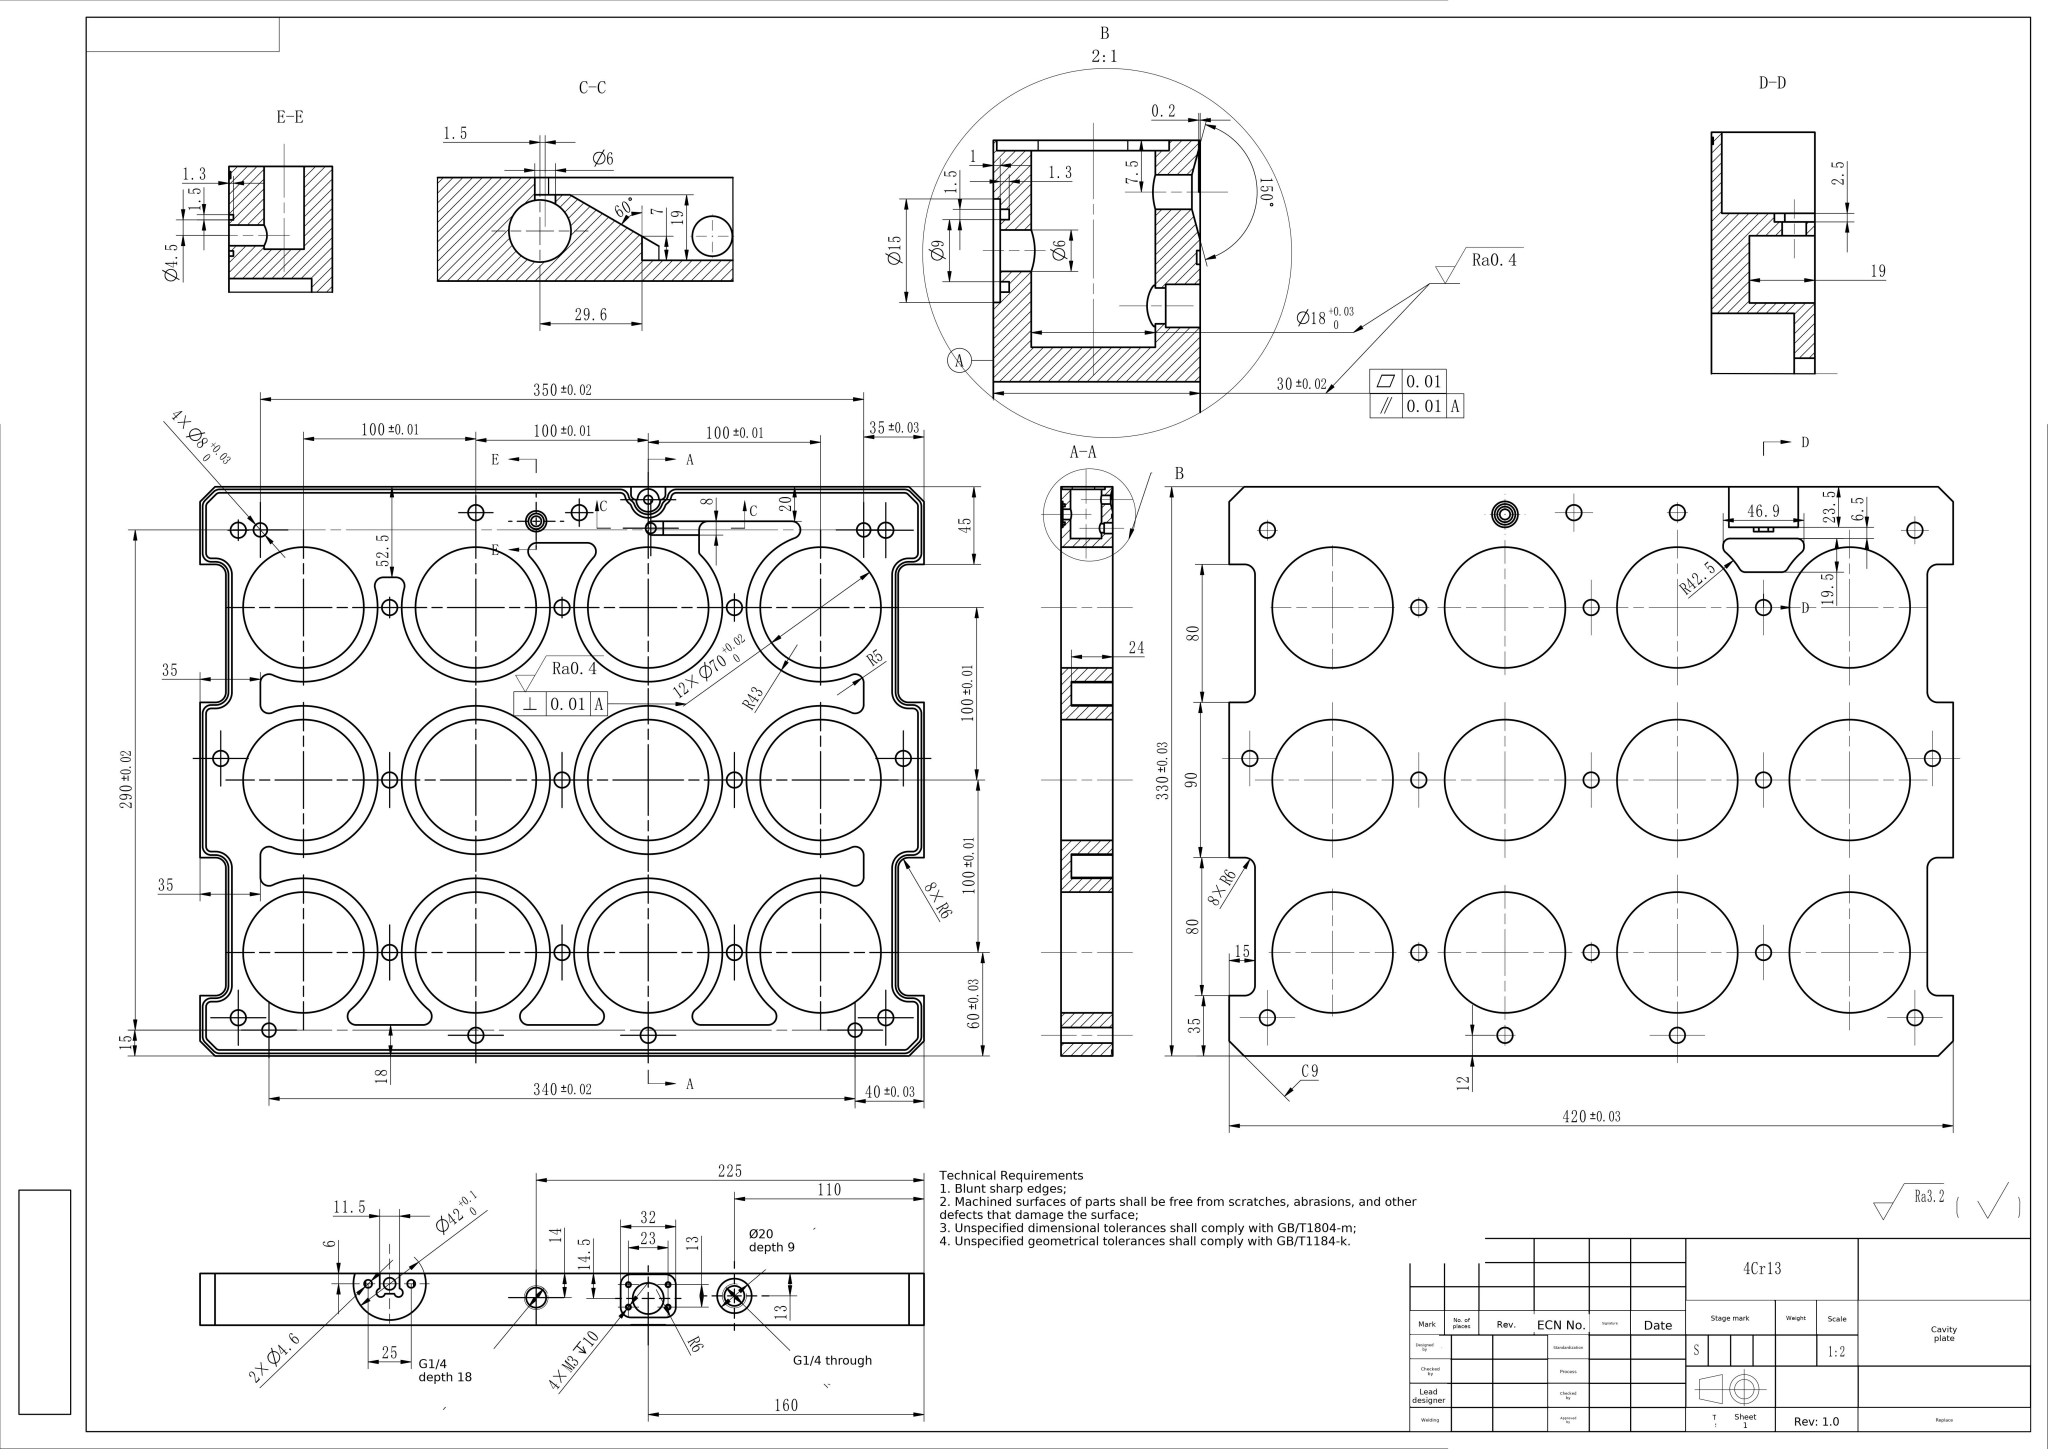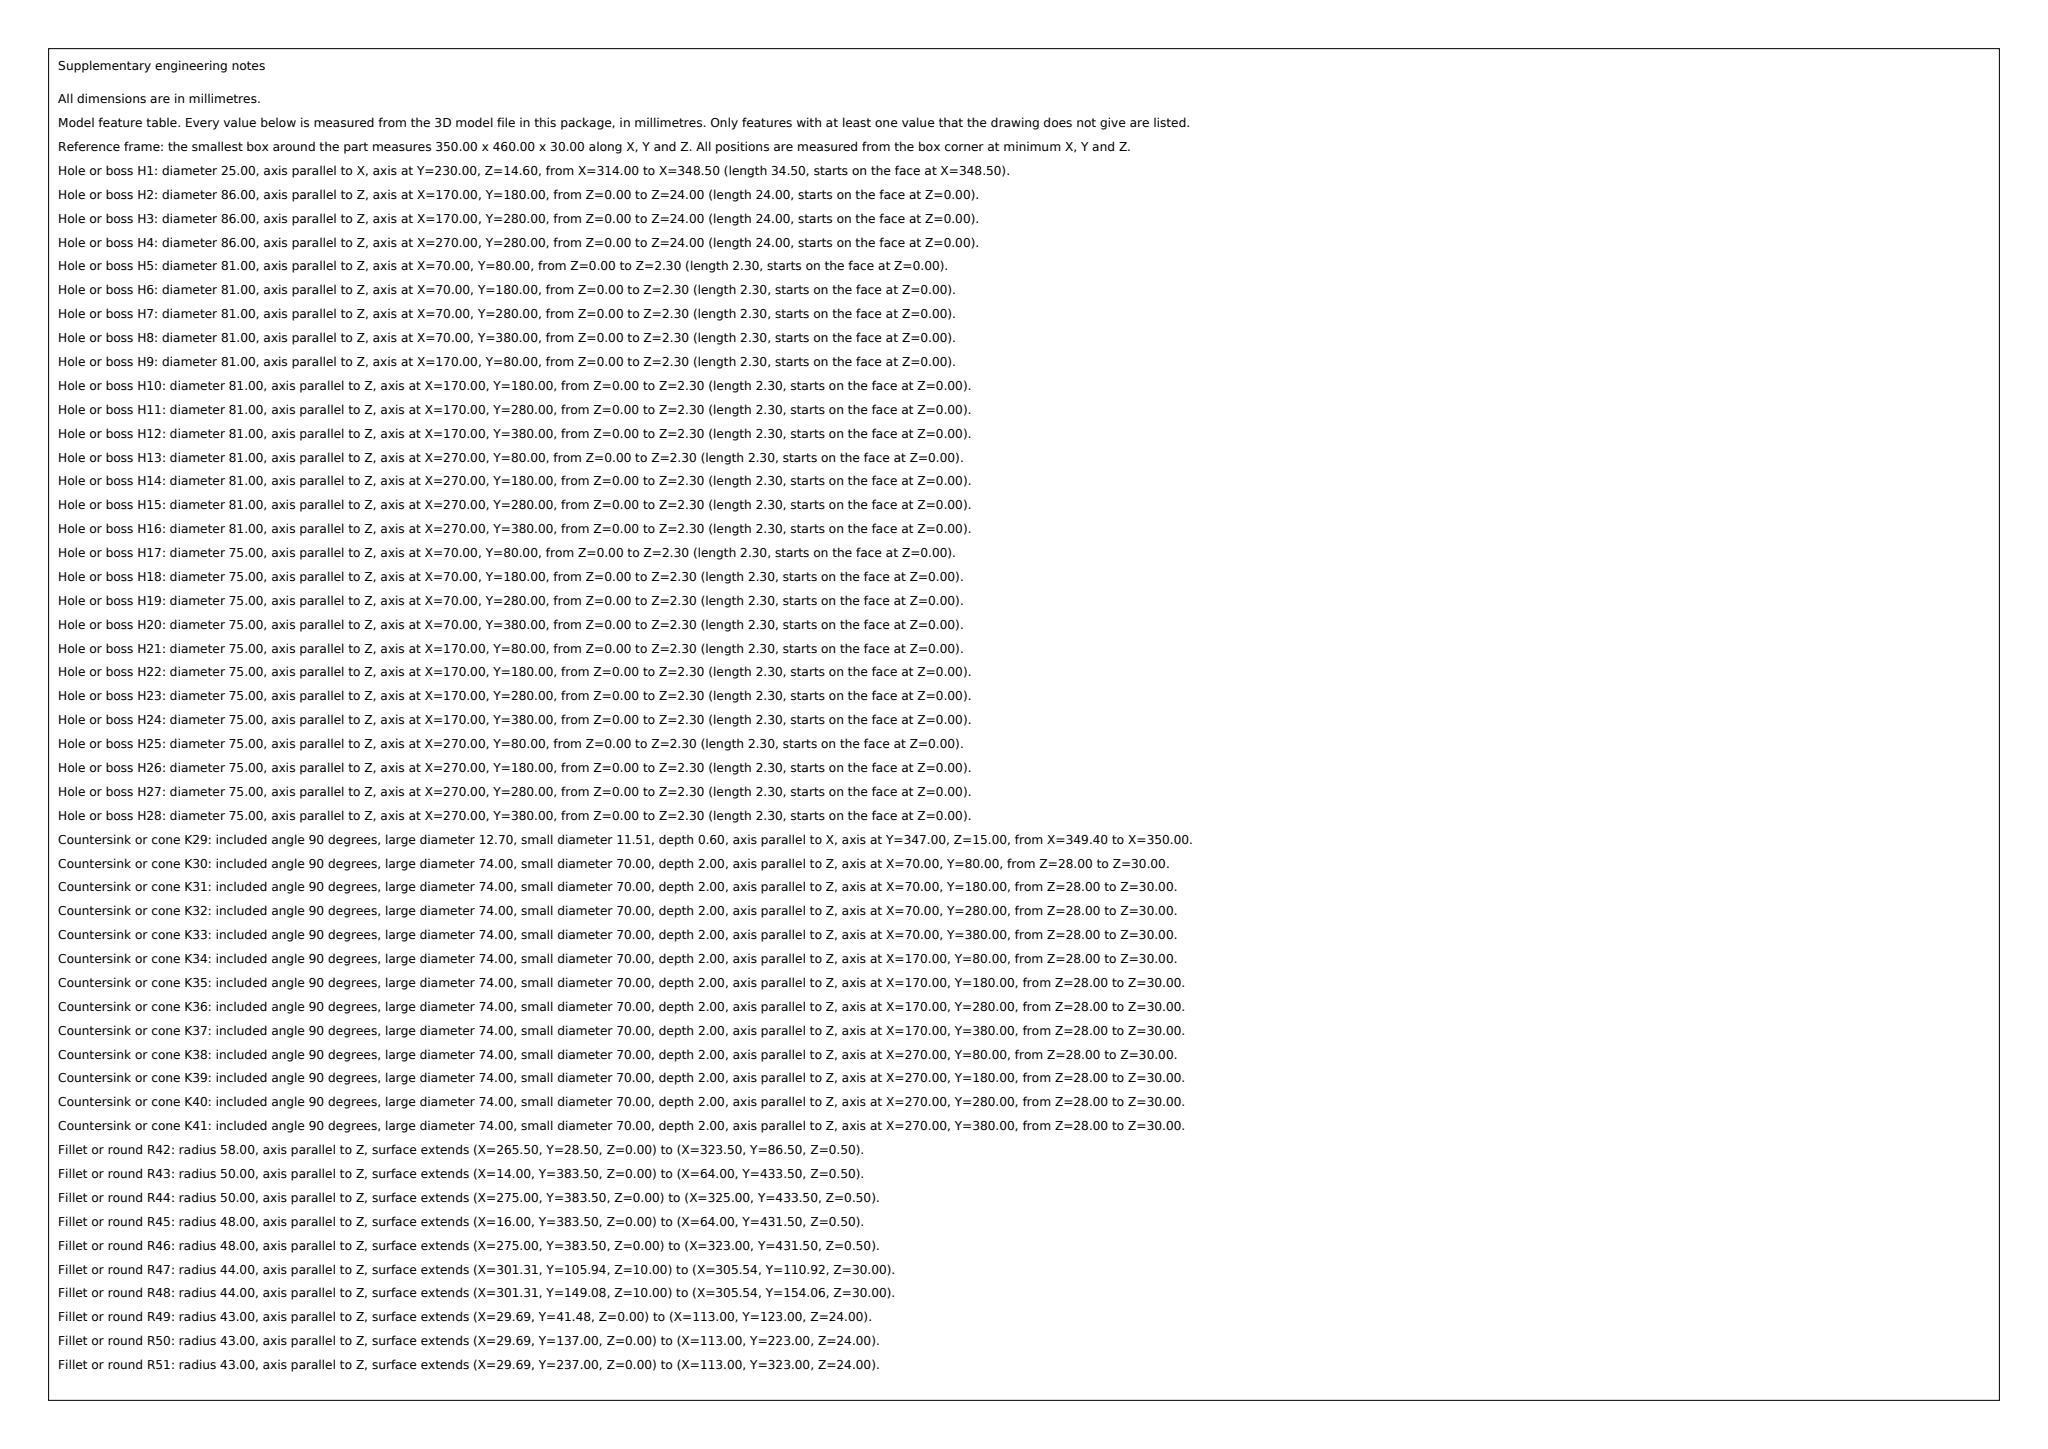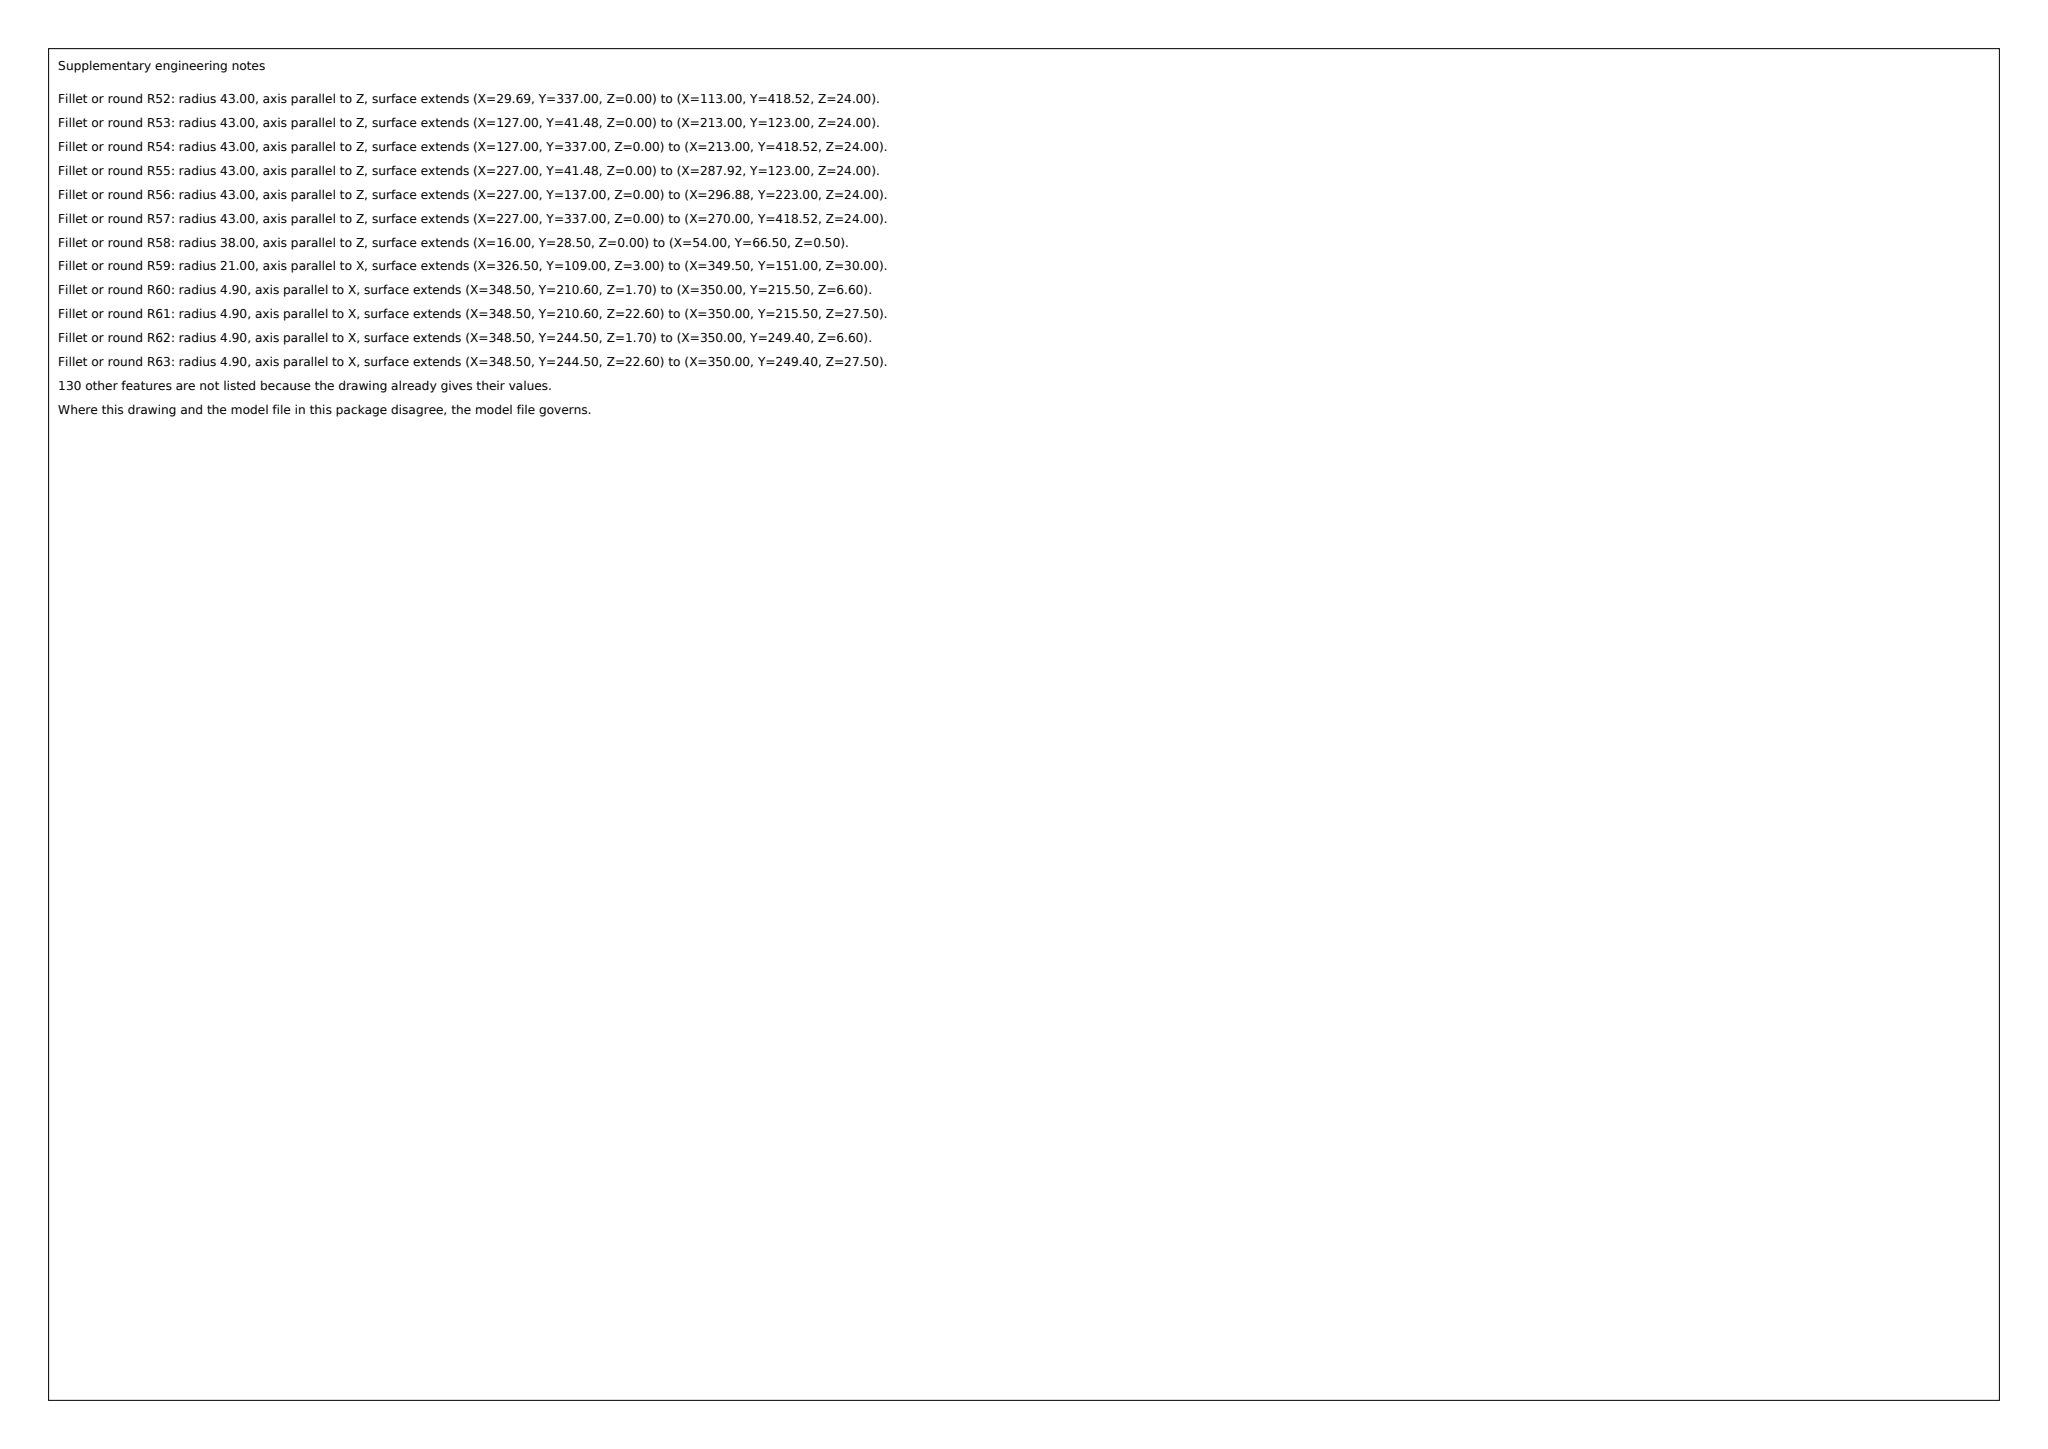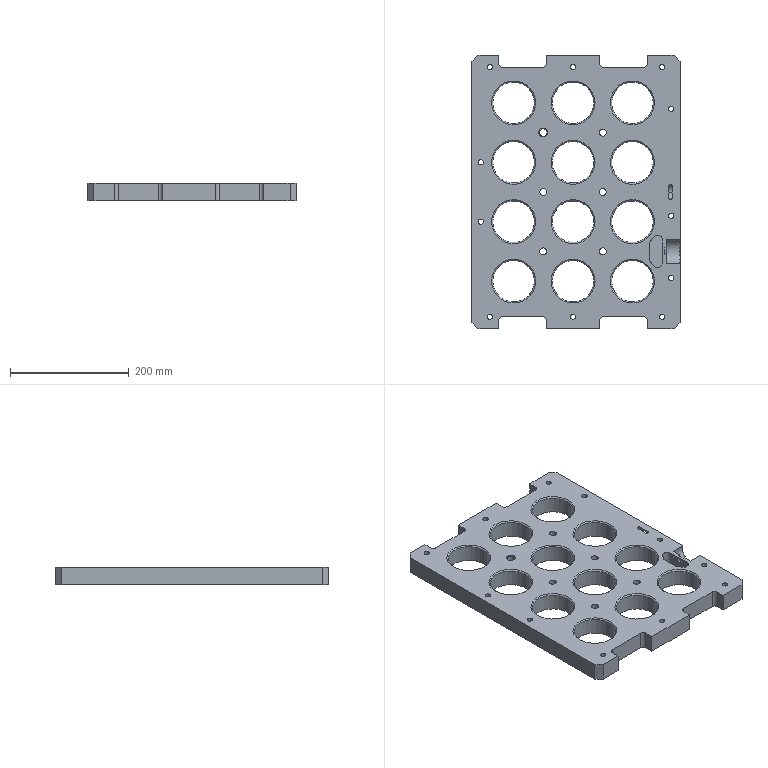Part | SolidWorks | mm | material 4Cr13 | 1 solid | 445 faces | box 350 x 460 x 30 mm | volume 2159804 mm3 | cylinder 273 | plane 126 | cone 46 | commonest cylinder face diameters 10 x33 75 x24 81 x24 9 x24 12 x24 70 x24 86 x23 20 x21